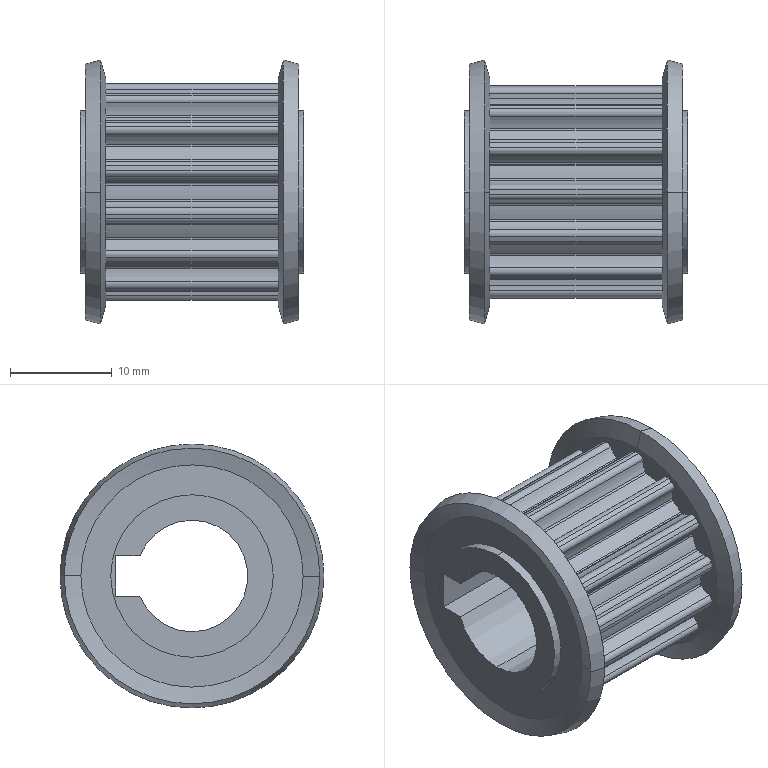Component | SolidWorks | EBJ22-S5M150-14-A-H-d10-3 | 1 solid | 153 faces | volume 4675 mm3 | cylinder 132 | cone 12 | plane 9 | commonest cylinder face diameters 1.1 x34 0.5 x32 6.55 x30 21.32 x15 17.78 x14 16 x4 11 x3